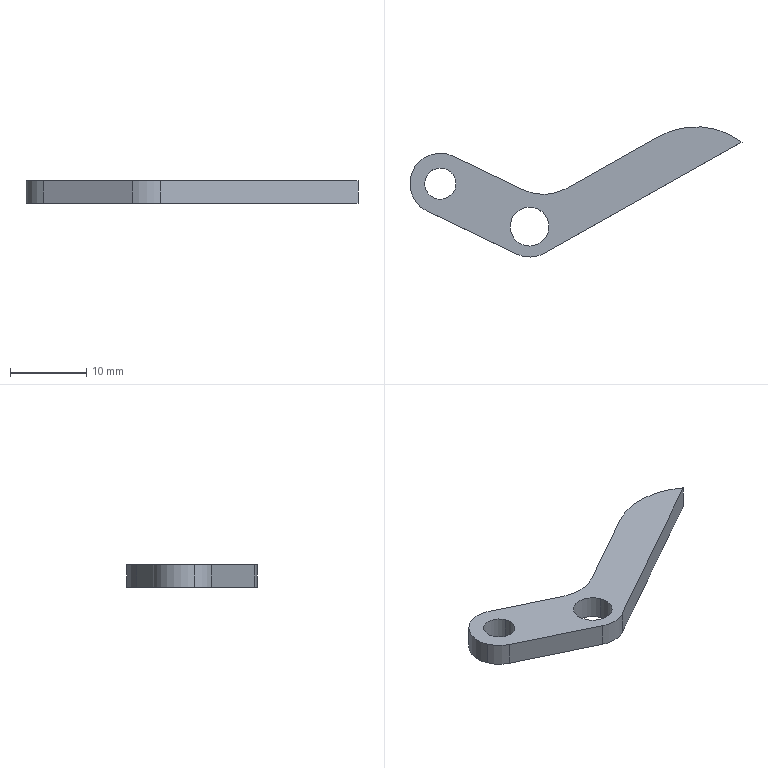Component | SolidWorks | JR-PL-JD-15Scissors-1 | 1 solid | 15 faces | box 43.6 x 17.1 x 3 mm | volume 795 mm3 | cylinder 9 | plane 6 | commonest cylinder face diameters 8 x3 4.1 x2 5.1 x2 12 x1 20 x1
build123d program:
from build123d import *

# Parameters (mm, degrees)
SKETCH1_R           = 2.55
SKETCH1_R_2         = 2.05
BOSS_EXTRUDE1_DEPTH = 3


with BuildPart() as part:
    # Sketch1 → Boss-Extrude1 (new body)
    with BuildSketch(Plane.XY):
        with BuildLine():
            Line((-2.941, -2.711), (-11.751, 6.849))
            ThreePointArc((-11.751, 6.849), (-11.52, 12.501), (-5.868, 12.27))
            Line((-5.868, 12.27), (1.068, 4.743))
            ThreePointArc((1.068, 4.743), (3.444, 3.165), (6.28, 2.863))
            Line((6.28, 2.863), (20.117, 4.724))
            ThreePointArc((20.117, 4.724), (25.763, 3.836), (30, 0))
            Line((30, 0), (0.5333, -3.964))
            ThreePointArc((0.5333, -3.964), (-1.357, -3.763), (-2.941, -2.711))
        make_face()
        Circle(SKETCH1_R, mode=Mode.SUBTRACT)
        with Locations((-8.81, 9.56)):
            Circle(SKETCH1_R_2, mode=Mode.SUBTRACT)
    extrude(amount=BOSS_EXTRUDE1_DEPTH)


solid = part.part

# Placed as in the assembly
solid = solid.moved(Location((37.675, 30.452, 70.77), (0, 0, 21.679)))
STEP:
#1=CARTESIAN_POINT('',(0.9469,1.391,2.904));
#2=VERTEX_POINT('',#1);
#3=CARTESIAN_POINT('',(1.097,1.45,2.904));
#4=VERTEX_POINT('',#3);
#5=CARTESIAN_POINT('',(1.022,1.421,2.904));
#6=DIRECTION('',(-0.,0.,1.));
#7=DIRECTION('',(0.9293,0.3694,0.));
#8=AXIS2_PLACEMENT_3D('',#5,#6,#7);
#9=CIRCLE('',#8,0.08071);
#10=EDGE_CURVE('',#2,#4,#9,.T.);
#11=ORIENTED_EDGE('',*,*,#10,.T.);
#12=CARTESIAN_POINT('',(1.097,1.45,2.786));
#13=VERTEX_POINT('',#12);
#14=CARTESIAN_POINT('',(1.097,1.45,2.904));
#15=DIRECTION('',(0.,-0.,-1.));
#16=VECTOR('',#15,39.37);
#17=LINE('',#14,#16);
#18=EDGE_CURVE('',#4,#13,#17,.T.);
#19=ORIENTED_EDGE('',*,*,#18,.T.);
#20=CARTESIAN_POINT('',(0.9469,1.391,2.786));
#21=VERTEX_POINT('',#20);
#22=CARTESIAN_POINT('',(1.022,1.421,2.786));
#23=DIRECTION('',(-0.,0.,1.));
#24=DIRECTION('',(0.9293,0.3694,0.));
#25=AXIS2_PLACEMENT_3D('',#22,#23,#24);
#26=CIRCLE('',#25,0.08071);
#27=EDGE_CURVE('',#21,#13,#26,.T.);
#28=ORIENTED_EDGE('',*,*,#27,.F.);
#29=CARTESIAN_POINT('',(0.9469,1.391,2.904));
#30=DIRECTION('',(0.,-0.,-1.));
#31=VECTOR('',#30,39.37);
#32=LINE('',#29,#31);
#33=EDGE_CURVE('',#2,#21,#32,.T.);
#34=ORIENTED_EDGE('',*,*,#33,.F.);
#35=EDGE_LOOP('',(#11,#19,#28,#34));
#36=FACE_OUTER_BOUND('',#35,.T.);
#37=CARTESIAN_POINT('',(1.022,1.421,2.904));
#38=DIRECTION('',(0.,-0.,-1.));
#39=DIRECTION('',(-0.9293,-0.3694,0.));
#40=AXIS2_PLACEMENT_3D('',#37,#38,#39);
#41=CYLINDRICAL_SURFACE('',#40,0.08071);
#42=ADVANCED_FACE('',(#36),#41,.F.);
#43=CARTESIAN_POINT('',(1.39,1.162,2.904));
#44=VERTEX_POINT('',#43);
#45=CARTESIAN_POINT('',(1.577,1.236,2.904));
#46=VERTEX_POINT('',#45);
#47=CARTESIAN_POINT('',(1.483,1.199,2.904));
#48=DIRECTION('',(-0.,0.,1.));
#49=DIRECTION('',(0.9293,0.3694,0.));
#50=AXIS2_PLACEMENT_3D('',#47,#48,#49);
#51=CIRCLE('',#50,0.1004);
#52=EDGE_CURVE('',#44,#46,#51,.T.);
#53=ORIENTED_EDGE('',*,*,#52,.T.);
#54=CARTESIAN_POINT('',(1.577,1.236,2.786));
#55=VERTEX_POINT('',#54);
#56=CARTESIAN_POINT('',(1.577,1.236,2.904));
#57=DIRECTION('',(0.,-0.,-1.));
#58=VECTOR('',#57,39.37);
#59=LINE('',#56,#58);
#60=EDGE_CURVE('',#46,#55,#59,.T.);
#61=ORIENTED_EDGE('',*,*,#60,.T.);
#62=CARTESIAN_POINT('',(1.39,1.162,2.786));
#63=VERTEX_POINT('',#62);
#64=CARTESIAN_POINT('',(1.483,1.199,2.786));
#65=DIRECTION('',(-0.,0.,1.));
#66=DIRECTION('',(0.9293,0.3694,0.));
#67=AXIS2_PLACEMENT_3D('',#64,#65,#66);
#68=CIRCLE('',#67,0.1004);
#69=EDGE_CURVE('',#63,#55,#68,.T.);
#70=ORIENTED_EDGE('',*,*,#69,.F.);
#71=CARTESIAN_POINT('',(1.39,1.162,2.904));
#72=DIRECTION('',(0.,-0.,-1.));
#73=VECTOR('',#72,39.37);
#74=LINE('',#71,#73);
#75=EDGE_CURVE('',#44,#63,#74,.T.);
#76=ORIENTED_EDGE('',*,*,#75,.F.);
#77=EDGE_LOOP('',(#53,#61,#70,#76));
#78=FACE_OUTER_BOUND('',#77,.T.);
#79=CARTESIAN_POINT('',(1.483,1.199,2.904));
#80=DIRECTION('',(0.,-0.,-1.));
#81=DIRECTION('',(-0.9293,-0.3694,0.));
#82=AXIS2_PLACEMENT_3D('',#79,#80,#81);
#83=CYLINDRICAL_SURFACE('',#82,0.1004);
#84=ADVANCED_FACE('',(#78),#83,.F.);
#85=CARTESIAN_POINT('',(0.8756,1.362,2.904));
#86=VERTEX_POINT('',#85);
#87=CARTESIAN_POINT('',(0.9537,1.279,2.904));
#88=VERTEX_POINT('',#87);
#89=CARTESIAN_POINT('',(1.022,1.421,2.904));
#90=DIRECTION('',(-0.,0.,1.));
#91=DIRECTION('',(0.9293,0.3694,0.));
#92=AXIS2_PLACEMENT_3D('',#89,#90,#91);
#93=CIRCLE('',#92,0.1575);
#94=EDGE_CURVE('',#86,#88,#93,.T.);
#95=ORIENTED_EDGE('',*,*,#94,.F.);
#96=CARTESIAN_POINT('',(0.8756,1.362,2.786));
#97=VERTEX_POINT('',#96);
#98=CARTESIAN_POINT('',(0.8756,1.362,2.904));
#99=DIRECTION('',(0.,-0.,-1.));
#100=VECTOR('',#99,39.37);
#101=LINE('',#98,#100);
#102=EDGE_CURVE('',#86,#97,#101,.T.);
#103=ORIENTED_EDGE('',*,*,#102,.T.);
#104=CARTESIAN_POINT('',(0.9537,1.279,2.786));
#105=VERTEX_POINT('',#104);
#106=CARTESIAN_POINT('',(1.022,1.421,2.786));
#107=DIRECTION('',(-0.,0.,1.));
#108=DIRECTION('',(0.9293,0.3694,0.));
#109=AXIS2_PLACEMENT_3D('',#106,#107,#108);
#110=CIRCLE('',#109,0.1575);
#111=EDGE_CURVE('',#97,#105,#110,.T.);
#112=ORIENTED_EDGE('',*,*,#111,.T.);
#113=CARTESIAN_POINT('',(0.9537,1.279,2.904));
#114=DIRECTION('',(0.,-0.,-1.));
#115=VECTOR('',#114,39.37);
#116=LINE('',#113,#115);
#117=EDGE_CURVE('',#88,#105,#116,.T.);
#118=ORIENTED_EDGE('',*,*,#117,.F.);
#119=EDGE_LOOP('',(#95,#103,#112,#118));
#120=FACE_OUTER_BOUND('',#119,.T.);
#121=CARTESIAN_POINT('',(1.022,1.421,2.904));
#122=DIRECTION('',(0.,-0.,-1.));
#123=DIRECTION('',(-0.9293,-0.3694,0.));
#124=AXIS2_PLACEMENT_3D('',#121,#122,#123);
#125=CYLINDRICAL_SURFACE('',#124,0.1575);
#126=ADVANCED_FACE('',(#120),#125,.T.);
#127=CARTESIAN_POINT('',(1.671,1.395,2.904));
#128=VERTEX_POINT('',#127);
#129=CARTESIAN_POINT('',(1.453,1.388,2.904));
#130=VERTEX_POINT('',#129);
#131=CARTESIAN_POINT('',(1.556,1.601,2.904));
#132=DIRECTION('',(0.,-0.,-1.));
#133=DIRECTION('',(-0.9293,-0.3694,0.));
#134=AXIS2_PLACEMENT_3D('',#131,#132,#133);
#135=CIRCLE('',#134,0.2362);
#136=EDGE_CURVE('',#128,#130,#135,.T.);
#137=ORIENTED_EDGE('',*,*,#136,.T.);
#138=CARTESIAN_POINT('',(1.09,1.562,2.904));
#139=VERTEX_POINT('',#138);
#140=CARTESIAN_POINT('',(1.453,1.388,2.904));
#141=DIRECTION('',(-0.9014,0.433,-0.));
#142=VECTOR('',#141,39.37);
#143=LINE('',#140,#142);
#144=EDGE_CURVE('',#130,#139,#143,.T.);
#145=ORIENTED_EDGE('',*,*,#144,.T.);
#146=CARTESIAN_POINT('',(1.022,1.421,2.904));
#147=DIRECTION('',(-0.,0.,1.));
#148=DIRECTION('',(0.9293,0.3694,0.));
#149=AXIS2_PLACEMENT_3D('',#146,#147,#148);
#150=CIRCLE('',#149,0.1575);
#151=EDGE_CURVE('',#139,#86,#150,.T.);
#152=ORIENTED_EDGE('',*,*,#151,.T.);
#153=ORIENTED_EDGE('',*,*,#94,.T.);
#154=CARTESIAN_POINT('',(1.415,1.057,2.904));
#155=VERTEX_POINT('',#154);
#156=CARTESIAN_POINT('',(1.415,1.057,2.904));
#157=DIRECTION('',(0.9014,-0.433,0.));
#158=VECTOR('',#157,39.37);
#159=LINE('',#156,#158);
#160=EDGE_CURVE('',#88,#155,#159,.T.);
#161=ORIENTED_EDGE('',*,*,#160,.T.);
#162=CARTESIAN_POINT('',(1.56,1.062,2.904));
#163=VERTEX_POINT('',#162);
#164=CARTESIAN_POINT('',(1.483,1.199,2.904));
#165=DIRECTION('',(-0.,0.,1.));
#166=DIRECTION('',(0.9293,0.3694,0.));
#167=AXIS2_PLACEMENT_3D('',#164,#165,#166);
#168=CIRCLE('',#167,0.1575);
#169=EDGE_CURVE('',#155,#163,#168,.T.);
#170=ORIENTED_EDGE('',*,*,#169,.T.);
#171=CARTESIAN_POINT('',(2.581,1.635,2.904));
#172=VERTEX_POINT('',#171);
#173=CARTESIAN_POINT('',(1.56,1.062,2.904));
#174=DIRECTION('',(0.8717,0.49,0.));
#175=VECTOR('',#174,39.37);
#176=LINE('',#173,#175);
#177=EDGE_CURVE('',#163,#172,#176,.T.);
#178=ORIENTED_EDGE('',*,*,#177,.T.);
#179=CARTESIAN_POINT('',(2.151,1.664,2.904));
#180=VERTEX_POINT('',#179);
#181=CARTESIAN_POINT('',(2.343,1.321,2.904));
#182=DIRECTION('',(-0.,0.,1.));
#183=DIRECTION('',(0.9293,0.3694,0.));
#184=AXIS2_PLACEMENT_3D('',#181,#182,#183);
#185=CIRCLE('',#184,0.3937);
#186=EDGE_CURVE('',#172,#180,#185,.T.);
#187=ORIENTED_EDGE('',*,*,#186,.T.);
#188=CARTESIAN_POINT('',(1.671,1.395,2.904));
#189=DIRECTION('',(-0.8717,-0.49,-0.));
#190=VECTOR('',#189,39.37);
#191=LINE('',#188,#190);
#192=EDGE_CURVE('',#180,#128,#191,.T.);
#193=ORIENTED_EDGE('',*,*,#192,.T.);
#194=EDGE_LOOP('',(#137,#145,#152,#153,#161,#170,#178,#187,#193));
#195=FACE_OUTER_BOUND('',#194,.T.);
#196=ORIENTED_EDGE('',*,*,#52,.F.);
#197=CARTESIAN_POINT('',(1.483,1.199,2.904));
#198=DIRECTION('',(-0.,0.,1.));
#199=DIRECTION('',(0.9293,0.3694,0.));
#200=AXIS2_PLACEMENT_3D('',#197,#198,#199);
#201=CIRCLE('',#200,0.1004);
#202=EDGE_CURVE('',#46,#44,#201,.T.);
#203=ORIENTED_EDGE('',*,*,#202,.F.);
#204=EDGE_LOOP('',(#196,#203));
#205=FACE_BOUND('',#204,.T.);
#206=ORIENTED_EDGE('',*,*,#10,.F.);
#207=CARTESIAN_POINT('',(1.022,1.421,2.904));
#208=DIRECTION('',(-0.,0.,1.));
#209=DIRECTION('',(0.9293,0.3694,0.));
#210=AXIS2_PLACEMENT_3D('',#207,#208,#209);
#211=CIRCLE('',#210,0.08071);
#212=EDGE_CURVE('',#4,#2,#211,.T.);
#213=ORIENTED_EDGE('',*,*,#212,.F.);
#214=EDGE_LOOP('',(#206,#213));
#215=FACE_BOUND('',#214,.T.);
#216=CARTESIAN_POINT('',(1.556,1.601,2.904));
#217=DIRECTION('',(0.,-0.,-1.));
#218=DIRECTION('',(-0.9293,-0.3694,-0.));
#219=AXIS2_PLACEMENT_3D('',#216,#217,#218);
#220=PLANE('',#219);
#221=ADVANCED_FACE('',(#195,#205,#215),#220,.F.);
#222=ORIENTED_EDGE('',*,*,#69,.T.);
#223=CARTESIAN_POINT('',(1.483,1.199,2.786));
#224=DIRECTION('',(-0.,0.,1.));
#225=DIRECTION('',(0.9293,0.3694,0.));
#226=AXIS2_PLACEMENT_3D('',#223,#224,#225);
#227=CIRCLE('',#226,0.1004);
#228=EDGE_CURVE('',#55,#63,#227,.T.);
#229=ORIENTED_EDGE('',*,*,#228,.T.);
#230=EDGE_LOOP('',(#222,#229));
#231=FACE_BOUND('',#230,.T.);
#232=CARTESIAN_POINT('',(1.671,1.395,2.786));
#233=VERTEX_POINT('',#232);
#234=CARTESIAN_POINT('',(1.453,1.388,2.786));
#235=VERTEX_POINT('',#234);
#236=CARTESIAN_POINT('',(1.556,1.601,2.786));
#237=DIRECTION('',(0.,-0.,-1.));
#238=DIRECTION('',(-0.9293,-0.3694,0.));
#239=AXIS2_PLACEMENT_3D('',#236,#237,#238);
#240=CIRCLE('',#239,0.2362);
#241=EDGE_CURVE('',#233,#235,#240,.T.);
#242=ORIENTED_EDGE('',*,*,#241,.F.);
#243=CARTESIAN_POINT('',(2.151,1.664,2.786));
#244=VERTEX_POINT('',#243);
#245=CARTESIAN_POINT('',(1.671,1.395,2.786));
#246=DIRECTION('',(-0.8717,-0.49,-0.));
#247=VECTOR('',#246,39.37);
#248=LINE('',#245,#247);
#249=EDGE_CURVE('',#244,#233,#248,.T.);
#250=ORIENTED_EDGE('',*,*,#249,.F.);
#251=CARTESIAN_POINT('',(2.581,1.635,2.786));
#252=VERTEX_POINT('',#251);
#253=CARTESIAN_POINT('',(2.343,1.321,2.786));
#254=DIRECTION('',(-0.,0.,1.));
#255=DIRECTION('',(0.9293,0.3694,0.));
#256=AXIS2_PLACEMENT_3D('',#253,#254,#255);
#257=CIRCLE('',#256,0.3937);
#258=EDGE_CURVE('',#252,#244,#257,.T.);
#259=ORIENTED_EDGE('',*,*,#258,.F.);
#260=CARTESIAN_POINT('',(1.56,1.062,2.786));
#261=VERTEX_POINT('',#260);
#262=CARTESIAN_POINT('',(1.56,1.062,2.786));
#263=DIRECTION('',(0.8717,0.49,0.));
#264=VECTOR('',#263,39.37);
#265=LINE('',#262,#264);
#266=EDGE_CURVE('',#261,#252,#265,.T.);
#267=ORIENTED_EDGE('',*,*,#266,.F.);
#268=CARTESIAN_POINT('',(1.415,1.057,2.786));
#269=VERTEX_POINT('',#268);
#270=CARTESIAN_POINT('',(1.483,1.199,2.786));
#271=DIRECTION('',(-0.,0.,1.));
#272=DIRECTION('',(0.9293,0.3694,0.));
#273=AXIS2_PLACEMENT_3D('',#270,#271,#272);
#274=CIRCLE('',#273,0.1575);
#275=EDGE_CURVE('',#269,#261,#274,.T.);
#276=ORIENTED_EDGE('',*,*,#275,.F.);
#277=CARTESIAN_POINT('',(1.415,1.057,2.786));
#278=DIRECTION('',(0.9014,-0.433,0.));
#279=VECTOR('',#278,39.37);
#280=LINE('',#277,#279);
#281=EDGE_CURVE('',#105,#269,#280,.T.);
#282=ORIENTED_EDGE('',*,*,#281,.F.);
#283=ORIENTED_EDGE('',*,*,#111,.F.);
#284=CARTESIAN_POINT('',(1.09,1.562,2.786));
#285=VERTEX_POINT('',#284);
#286=CARTESIAN_POINT('',(1.022,1.421,2.786));
#287=DIRECTION('',(-0.,0.,1.));
#288=DIRECTION('',(0.9293,0.3694,0.));
#289=AXIS2_PLACEMENT_3D('',#286,#287,#288);
#290=CIRCLE('',#289,0.1575);
#291=EDGE_CURVE('',#285,#97,#290,.T.);
#292=ORIENTED_EDGE('',*,*,#291,.F.);
#293=CARTESIAN_POINT('',(1.453,1.388,2.786));
#294=DIRECTION('',(-0.9014,0.433,-0.));
#295=VECTOR('',#294,39.37);
#296=LINE('',#293,#295);
#297=EDGE_CURVE('',#235,#285,#296,.T.);
#298=ORIENTED_EDGE('',*,*,#297,.F.);
#299=EDGE_LOOP('',(#242,#250,#259,#267,#276,#282,#283,#292,#298));
#300=FACE_OUTER_BOUND('',#299,.T.);
#301=ORIENTED_EDGE('',*,*,#27,.T.);
#302=CARTESIAN_POINT('',(1.022,1.421,2.786));
#303=DIRECTION('',(-0.,0.,1.));
#304=DIRECTION('',(0.9293,0.3694,0.));
#305=AXIS2_PLACEMENT_3D('',#302,#303,#304);
#306=CIRCLE('',#305,0.08071);
#307=EDGE_CURVE('',#13,#21,#306,.T.);
#308=ORIENTED_EDGE('',*,*,#307,.T.);
#309=EDGE_LOOP('',(#301,#308));
#310=FACE_BOUND('',#309,.T.);
#311=CARTESIAN_POINT('',(1.556,1.601,2.786));
#312=DIRECTION('',(0.,-0.,-1.));
#313=DIRECTION('',(-0.9293,-0.3694,-0.));
#314=AXIS2_PLACEMENT_3D('',#311,#312,#313);
#315=PLANE('',#314);
#316=ADVANCED_FACE('',(#231,#300,#310),#315,.T.);
#317=ORIENTED_EDGE('',*,*,#241,.T.);
#318=CARTESIAN_POINT('',(1.453,1.388,2.904));
#319=DIRECTION('',(0.,-0.,-1.));
#320=VECTOR('',#319,39.37);
#321=LINE('',#318,#320);
#322=EDGE_CURVE('',#130,#235,#321,.T.);
#323=ORIENTED_EDGE('',*,*,#322,.F.);
#324=ORIENTED_EDGE('',*,*,#136,.F.);
#325=CARTESIAN_POINT('',(1.671,1.395,2.904));
#326=DIRECTION('',(0.,-0.,-1.));
#327=VECTOR('',#326,39.37);
#328=LINE('',#325,#327);
#329=EDGE_CURVE('',#128,#233,#328,.T.);
#330=ORIENTED_EDGE('',*,*,#329,.T.);
#331=EDGE_LOOP('',(#317,#323,#324,#330));
#332=FACE_OUTER_BOUND('',#331,.T.);
#333=CARTESIAN_POINT('',(1.556,1.601,2.904));
#334=DIRECTION('',(0.,-0.,-1.));
#335=DIRECTION('',(-0.9293,-0.3694,0.));
#336=AXIS2_PLACEMENT_3D('',#333,#334,#335);
#337=CYLINDRICAL_SURFACE('',#336,0.2362);
#338=ADVANCED_FACE('',(#332),#337,.F.);
#339=ORIENTED_EDGE('',*,*,#297,.T.);
#340=CARTESIAN_POINT('',(1.09,1.562,2.904));
#341=DIRECTION('',(0.,-0.,-1.));
#342=VECTOR('',#341,39.37);
#343=LINE('',#340,#342);
#344=EDGE_CURVE('',#139,#285,#343,.T.);
#345=ORIENTED_EDGE('',*,*,#344,.F.);
#346=ORIENTED_EDGE('',*,*,#144,.F.);
#347=ORIENTED_EDGE('',*,*,#322,.T.);
#348=EDGE_LOOP('',(#339,#345,#346,#347));
#349=FACE_OUTER_BOUND('',#348,.T.);
#350=CARTESIAN_POINT('',(1.453,1.388,2.904));
#351=DIRECTION('',(-0.433,-0.9014,0.));
#352=DIRECTION('',(0.9014,-0.433,0.));
#353=AXIS2_PLACEMENT_3D('',#350,#351,#352);
#354=PLANE('',#353);
#355=ADVANCED_FACE('',(#349),#354,.F.);
#356=ORIENTED_EDGE('',*,*,#102,.F.);
#357=ORIENTED_EDGE('',*,*,#151,.F.);
#358=ORIENTED_EDGE('',*,*,#344,.T.);
#359=ORIENTED_EDGE('',*,*,#291,.T.);
#360=EDGE_LOOP('',(#356,#357,#358,#359));
#361=FACE_OUTER_BOUND('',#360,.T.);
#362=CARTESIAN_POINT('',(1.022,1.421,2.904));
#363=DIRECTION('',(0.,-0.,-1.));
#364=DIRECTION('',(-0.9293,-0.3694,0.));
#365=AXIS2_PLACEMENT_3D('',#362,#363,#364);
#366=CYLINDRICAL_SURFACE('',#365,0.1575);
#367=ADVANCED_FACE('',(#361),#366,.T.);
#368=ORIENTED_EDGE('',*,*,#281,.T.);
#369=CARTESIAN_POINT('',(1.415,1.057,2.904));
#370=DIRECTION('',(0.,-0.,-1.));
#371=VECTOR('',#370,39.37);
#372=LINE('',#369,#371);
#373=EDGE_CURVE('',#155,#269,#372,.T.);
#374=ORIENTED_EDGE('',*,*,#373,.F.);
#375=ORIENTED_EDGE('',*,*,#160,.F.);
#376=ORIENTED_EDGE('',*,*,#117,.T.);
#377=EDGE_LOOP('',(#368,#374,#375,#376));
#378=FACE_OUTER_BOUND('',#377,.T.);
#379=CARTESIAN_POINT('',(1.415,1.057,2.904));
#380=DIRECTION('',(0.433,0.9014,-0.));
#381=DIRECTION('',(-0.9014,0.433,-0.));
#382=AXIS2_PLACEMENT_3D('',#379,#380,#381);
#383=PLANE('',#382);
#384=ADVANCED_FACE('',(#378),#383,.F.);
#385=ORIENTED_EDGE('',*,*,#275,.T.);
#386=CARTESIAN_POINT('',(1.56,1.062,2.904));
#387=DIRECTION('',(0.,-0.,-1.));
#388=VECTOR('',#387,39.37);
#389=LINE('',#386,#388);
#390=EDGE_CURVE('',#163,#261,#389,.T.);
#391=ORIENTED_EDGE('',*,*,#390,.F.);
#392=ORIENTED_EDGE('',*,*,#169,.F.);
#393=ORIENTED_EDGE('',*,*,#373,.T.);
#394=EDGE_LOOP('',(#385,#391,#392,#393));
#395=FACE_OUTER_BOUND('',#394,.T.);
#396=CARTESIAN_POINT('',(1.483,1.199,2.904));
#397=DIRECTION('',(0.,-0.,-1.));
#398=DIRECTION('',(-0.9293,-0.3694,0.));
#399=AXIS2_PLACEMENT_3D('',#396,#397,#398);
#400=CYLINDRICAL_SURFACE('',#399,0.1575);
#401=ADVANCED_FACE('',(#395),#400,.T.);
#402=ORIENTED_EDGE('',*,*,#266,.T.);
#403=CARTESIAN_POINT('',(2.581,1.635,2.904));
#404=DIRECTION('',(0.,-0.,-1.));
#405=VECTOR('',#404,39.37);
#406=LINE('',#403,#405);
#407=EDGE_CURVE('',#172,#252,#406,.T.);
#408=ORIENTED_EDGE('',*,*,#407,.F.);
#409=ORIENTED_EDGE('',*,*,#177,.F.);
#410=ORIENTED_EDGE('',*,*,#390,.T.);
#411=EDGE_LOOP('',(#402,#408,#409,#410));
#412=FACE_OUTER_BOUND('',#411,.T.);
#413=CARTESIAN_POINT('',(1.56,1.062,2.904));
#414=DIRECTION('',(-0.49,0.8717,-0.));
#415=DIRECTION('',(-0.8717,-0.49,-0.));
#416=AXIS2_PLACEMENT_3D('',#413,#414,#415);
#417=PLANE('',#416);
#418=ADVANCED_FACE('',(#412),#417,.F.);
#419=ORIENTED_EDGE('',*,*,#258,.T.);
#420=CARTESIAN_POINT('',(2.151,1.664,2.904));
#421=DIRECTION('',(0.,-0.,-1.));
#422=VECTOR('',#421,39.37);
#423=LINE('',#420,#422);
#424=EDGE_CURVE('',#180,#244,#423,.T.);
#425=ORIENTED_EDGE('',*,*,#424,.F.);
#426=ORIENTED_EDGE('',*,*,#186,.F.);
#427=ORIENTED_EDGE('',*,*,#407,.T.);
#428=EDGE_LOOP('',(#419,#425,#426,#427));
#429=FACE_OUTER_BOUND('',#428,.T.);
#430=CARTESIAN_POINT('',(2.343,1.321,2.904));
#431=DIRECTION('',(0.,-0.,-1.));
#432=DIRECTION('',(-0.9293,-0.3694,0.));
#433=AXIS2_PLACEMENT_3D('',#430,#431,#432);
#434=CYLINDRICAL_SURFACE('',#433,0.3937);
#435=ADVANCED_FACE('',(#429),#434,.T.);
#436=ORIENTED_EDGE('',*,*,#249,.T.);
#437=ORIENTED_EDGE('',*,*,#329,.F.);
#438=ORIENTED_EDGE('',*,*,#192,.F.);
#439=ORIENTED_EDGE('',*,*,#424,.T.);
#440=EDGE_LOOP('',(#436,#437,#438,#439));
#441=FACE_OUTER_BOUND('',#440,.T.);
#442=CARTESIAN_POINT('',(1.671,1.395,2.904));
#443=DIRECTION('',(0.49,-0.8717,0.));
#444=DIRECTION('',(0.8717,0.49,0.));
#445=AXIS2_PLACEMENT_3D('',#442,#443,#444);
#446=PLANE('',#445);
#447=ADVANCED_FACE('',(#441),#446,.F.);
#448=ORIENTED_EDGE('',*,*,#60,.F.);
#449=ORIENTED_EDGE('',*,*,#202,.T.);
#450=ORIENTED_EDGE('',*,*,#75,.T.);
#451=ORIENTED_EDGE('',*,*,#228,.F.);
#452=EDGE_LOOP('',(#448,#449,#450,#451));
#453=FACE_OUTER_BOUND('',#452,.T.);
#454=CARTESIAN_POINT('',(1.483,1.199,2.904));
#455=DIRECTION('',(0.,-0.,-1.));
#456=DIRECTION('',(-0.9293,-0.3694,0.));
#457=AXIS2_PLACEMENT_3D('',#454,#455,#456);
#458=CYLINDRICAL_SURFACE('',#457,0.1004);
#459=ADVANCED_FACE('',(#453),#458,.F.);
#460=ORIENTED_EDGE('',*,*,#18,.F.);
#461=ORIENTED_EDGE('',*,*,#212,.T.);
#462=ORIENTED_EDGE('',*,*,#33,.T.);
#463=ORIENTED_EDGE('',*,*,#307,.F.);
#464=EDGE_LOOP('',(#460,#461,#462,#463));
#465=FACE_OUTER_BOUND('',#464,.T.);
#466=CARTESIAN_POINT('',(1.022,1.421,2.904));
#467=DIRECTION('',(0.,-0.,-1.));
#468=DIRECTION('',(-0.9293,-0.3694,0.));
#469=AXIS2_PLACEMENT_3D('',#466,#467,#468);
#470=CYLINDRICAL_SURFACE('',#469,0.08071);
#471=ADVANCED_FACE('',(#465),#470,.F.);
#472=CLOSED_SHELL('',(#42,#84,#126,#221,#316,#338,#355,#367,#384,#401,#418,#435,#447,#459,#471));
#473=MANIFOLD_SOLID_BREP('',#472);
#474=CARTESIAN_POINT('',(0.,0.,0.));
#475=DIRECTION('',(0.,0.,1.));
#476=DIRECTION('',(1.,0.,0.));
#477=AXIS2_PLACEMENT_3D('',#474,#475,#476);
#478=(LENGTH_UNIT()NAMED_UNIT(*)SI_UNIT($,.METRE.));
#479=LENGTH_MEASURE_WITH_UNIT(LENGTH_MEASURE(0.0254),#478);
#480=DIMENSIONAL_EXPONENTS(1.,0.,0.,0.,0.,0.,0.);
#481=(CONVERSION_BASED_UNIT('',#479)LENGTH_UNIT()NAMED_UNIT(#480));
#482=UNCERTAINTY_MEASURE_WITH_UNIT(LENGTH_MEASURE(0.00001),#481,'','');
#483=(NAMED_UNIT(*)PLANE_ANGLE_UNIT()SI_UNIT($,.RADIAN.));
#484=(NAMED_UNIT(*)SI_UNIT($,.STERADIAN.)SOLID_ANGLE_UNIT());
#485=(GEOMETRIC_REPRESENTATION_CONTEXT(3)GLOBAL_UNCERTAINTY_ASSIGNED_CONTEXT((#482))GLOBAL_UNIT_ASSIGNED_CONTEXT((#481,#483,#484))REPRESENTATION_CONTEXT('',''));
#486=ADVANCED_BREP_SHAPE_REPRESENTATION('',(#473,#477),#485);
#487=COLOUR_RGB('',0.7922,0.8196,0.9333);
#488=FILL_AREA_STYLE_COLOUR('',#487);
#489=FILL_AREA_STYLE('',(#488));
#490=SURFACE_STYLE_FILL_AREA(#489);
#491=SURFACE_SIDE_STYLE('',(#490));
#492=SURFACE_STYLE_USAGE(.BOTH.,#491);
#493=PRESENTATION_STYLE_ASSIGNMENT((#492));
#494=STYLED_ITEM('',(#493),#473);
#495=(LENGTH_UNIT()NAMED_UNIT(*)SI_UNIT($,.METRE.));
#496=LENGTH_MEASURE_WITH_UNIT(LENGTH_MEASURE(0.0254),#495);
#497=DIMENSIONAL_EXPONENTS(1.,0.,0.,0.,0.,0.,0.);
#498=(CONVERSION_BASED_UNIT('',#496)LENGTH_UNIT()NAMED_UNIT(#497));
#499=UNCERTAINTY_MEASURE_WITH_UNIT(LENGTH_MEASURE(0.00001),#498,'','');
#500=(NAMED_UNIT(*)PLANE_ANGLE_UNIT()SI_UNIT($,.RADIAN.));
#501=(NAMED_UNIT(*)SI_UNIT($,.STERADIAN.)SOLID_ANGLE_UNIT());
#502=(GEOMETRIC_REPRESENTATION_CONTEXT(3)GLOBAL_UNCERTAINTY_ASSIGNED_CONTEXT((#499))GLOBAL_UNIT_ASSIGNED_CONTEXT((#498,#500,#501))REPRESENTATION_CONTEXT('',''));
#503=MECHANICAL_DESIGN_GEOMETRIC_PRESENTATION_REPRESENTATION('',(#494),#502);
#504=PRESENTATION_LAYER_ASSIGNMENT('','',(#494));